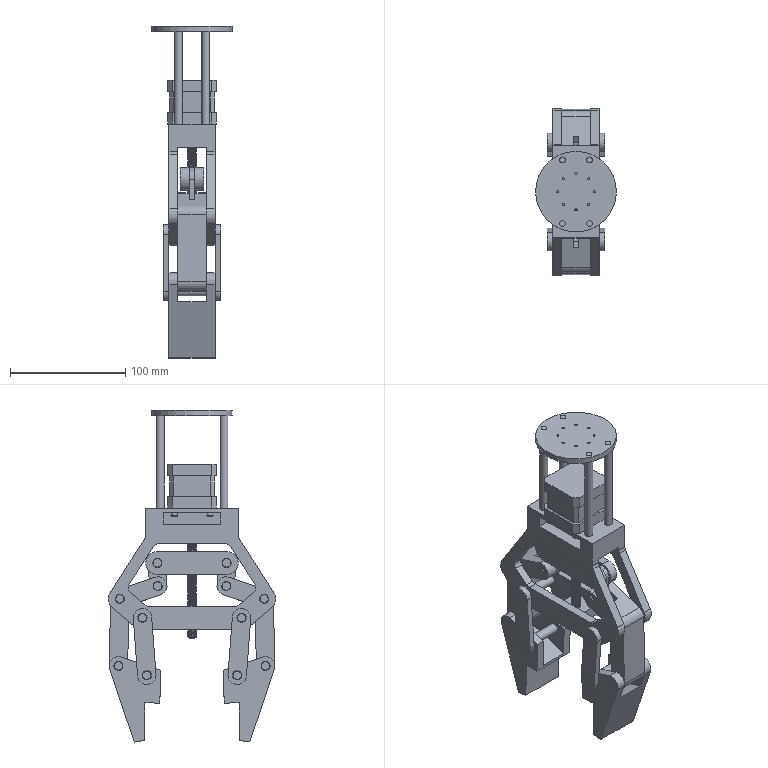Assembly | NX | mm | 35 component files | 35 solids | 503 faces | box 70 x 145 x 287.72 mm | volume 457254 mm3 | plane 254 | cylinder 160 | cone 77 | torus 8 | spline 4 | commonest cylinder face diameters 8 x56 16 x20 10 x18 5 x16 20 x12 2 x8 2.874 x4 5.5 x4
Bill of materials:
unnamed part 1 | 1 |  | Long, slender cylindrical rod with helical-looking thread ridges along its whole length and chamfered ends; no head (looks like a threaded rod or stud).
GB-T119.1-2000,8x50 | 4 |  | Parallel Pin, GB-T 119.1-2000,8x50
unnamed part 2 | 2 |  | Flat plate bent into an L or dog-leg shape, with rounded ends and three through-holes. One end is split by a slot into a two-tine clevis with a cross hole.
GB-T70.1-2000,M3x8 | 4 |  | Hexagon Socket Head Cap Screw, GB-T 70.1-2000,M3x8
GB-T119.1-2000,8x40 | 4 |  | Parallel Pin, GB-T 119.1-2000,8x40
unnamed part 3 | 2 |  | Short, thick flat link shaped like a stadium (obround), with two round through-holes near the rounded ends.
unnamed part 4 | 4 |  | Stepped cylindrical pin: a long main body with a shorter, smaller-diameter journal at each end.
unnamed part 5 | 1 |  | Bracket-like frame: a rectangular top block with a pattern of holes, carried on two parallel, trapezoid-shaped side plates with open windows. The side plates have pairs of holes near their lower corners, and a small cross tab with a hole spans between them near the bottom.
GB-T119.1-2000,8x26 | 2 |  | Parallel Pin, GB-T 119.1-2000,8x26
unnamed part 6 | 1 |  | Thin circular disc or plate with four larger holes near the rim and eight small holes on an inner circle.
unnamed part 7 | 2 |  | Clevis-style bracket: a solid base with two parallel, tapered ears that each have two through-holes, separated by a rectangular slot.
GB-T119.1-2000,8x20 | 2 |  | Parallel Pin, GB-T 119.1-2000,8x20
unnamed part 8 | 1 |  | Obround clevis link: two parallel rounded-end plates joined in the middle, with through-holes at both ends. Each end has a slot between the plates, and the center has a cross hole that looks threaded.
unnamed part 9 | 4 |  | Thin, slender flat link with rounded ends and two through-holes, one at each end.
unnamed part 10 | 1 |  | Square block with chamfered corners and a reduced-section groove around its middle, with a short shallow cylindrical boss on the underside.
Mates:
1. fix | Bracket 1 component
2. touch align | SimMotor 1 face | Bracket 1 face
3. touch align | SimMotor 1 face | Bracket 1 face
4. touch align | SimMotor 1 face | Bracket 1 face
5. concentric | LeadScrew 1 edge | Bracket 1 edge
6. touch align | PushPlate 1 face | LeadScrew 1 face
7. concentric | Link1 2 edge | PushPlate 1 edge
8. concentric | JawLink 2 edge | Link1 2 edge
9. concentric | JawLink2 4 edge | Bracket 1 edge
10. touch align | JawLink 2 face | Bracket 1 face
11. concentric | Jaw 2 edge | JawLink 2 edge
12. concentric | JawLink2 4 edge | Jaw 2 edge
13. concentric | JawLink2 3 edge | Bracket 1 edge
14. concentric | Jaw 2 edge | JawLink2 3 edge
15. concentric | Link1 1 edge | PushPlate 1 edge
16. concentric | JawLink 1 edge | Link1 1 edge
17. concentric | Bracket 1 edge | JawLink 1 edge
18. concentric | JawLink2 1 edge | Bracket 1 edge
19. concentric | JawLink2 2 edge | Bracket 1 edge
20. concentric | Jaw 1 edge | JawLink 1 edge
21. touch align | JawLink2 1 face | Jaw 1 face
22. touch align | JawLink2 2 face | Jaw 1 face
23. concentric | Strut 4 edge | Bracket 1 edge
24. concentric | Strut 3 edge | Bracket 1 edge
25. concentric | Strut 2 edge | Bracket 1 edge
26. concentric | Strut 1 edge | Bracket 1 edge
27. touch align | TopSeat 1 face | Strut 3 face
28. touch align | TopSeat 1 edge | Strut 2 face
29. touch align | TopSeat 1 face | Strut 4 face
30. concentric | GB-T119_1-2000_8x20 2 edge | PushPlate 1 edge
31. concentric | GB-T119_1-2000_8x26 2 edge | JawLink 2 edge
32. concentric | GB-T119_1-2000_8x40 4 edge | Bracket 1 edge
33. concentric | GB-T119_1-2000_8x50 4 edge | JawLink2 4 edge
34. concentric | GB-T119_1-2000_8x20 1 edge | PushPlate 1 edge
35. concentric | GB-T119_1-2000_8x26 1 edge | JawLink 1 edge
36. concentric | GB-T119_1-2000_8x40 2 edge | Bracket 1 edge
37. concentric | GB-T119_1-2000_8x40 1 edge | Jaw 1 edge
38. concentric | GB-T119_1-2000_8x40 3 edge | Jaw 2 edge
39. concentric | GB-T119_1-2000_8x50 1 edge | JawLink2 4 edge
40. concentric | GB-T119_1-2000_8x50 2 edge | JawLink2 1 edge
41. concentric | GB-T119_1-2000_8x50 3 edge | JawLink2 1 edge
42. concentric | GB-T119_1-2000_8x50 4 edge | JawLink2 4 edge
43. concentric | GB-T70_1-2000_M3x8 4 edge | Bracket 1 edge
44. concentric | GB-T70_1-2000_M3x8 3 edge | Bracket 1 edge
45. concentric | GB-T70_1-2000_M3x8 1 edge | Bracket 1 edge
46. concentric | GB-T70_1-2000_M3x8 2 edge | Bracket 1 edge